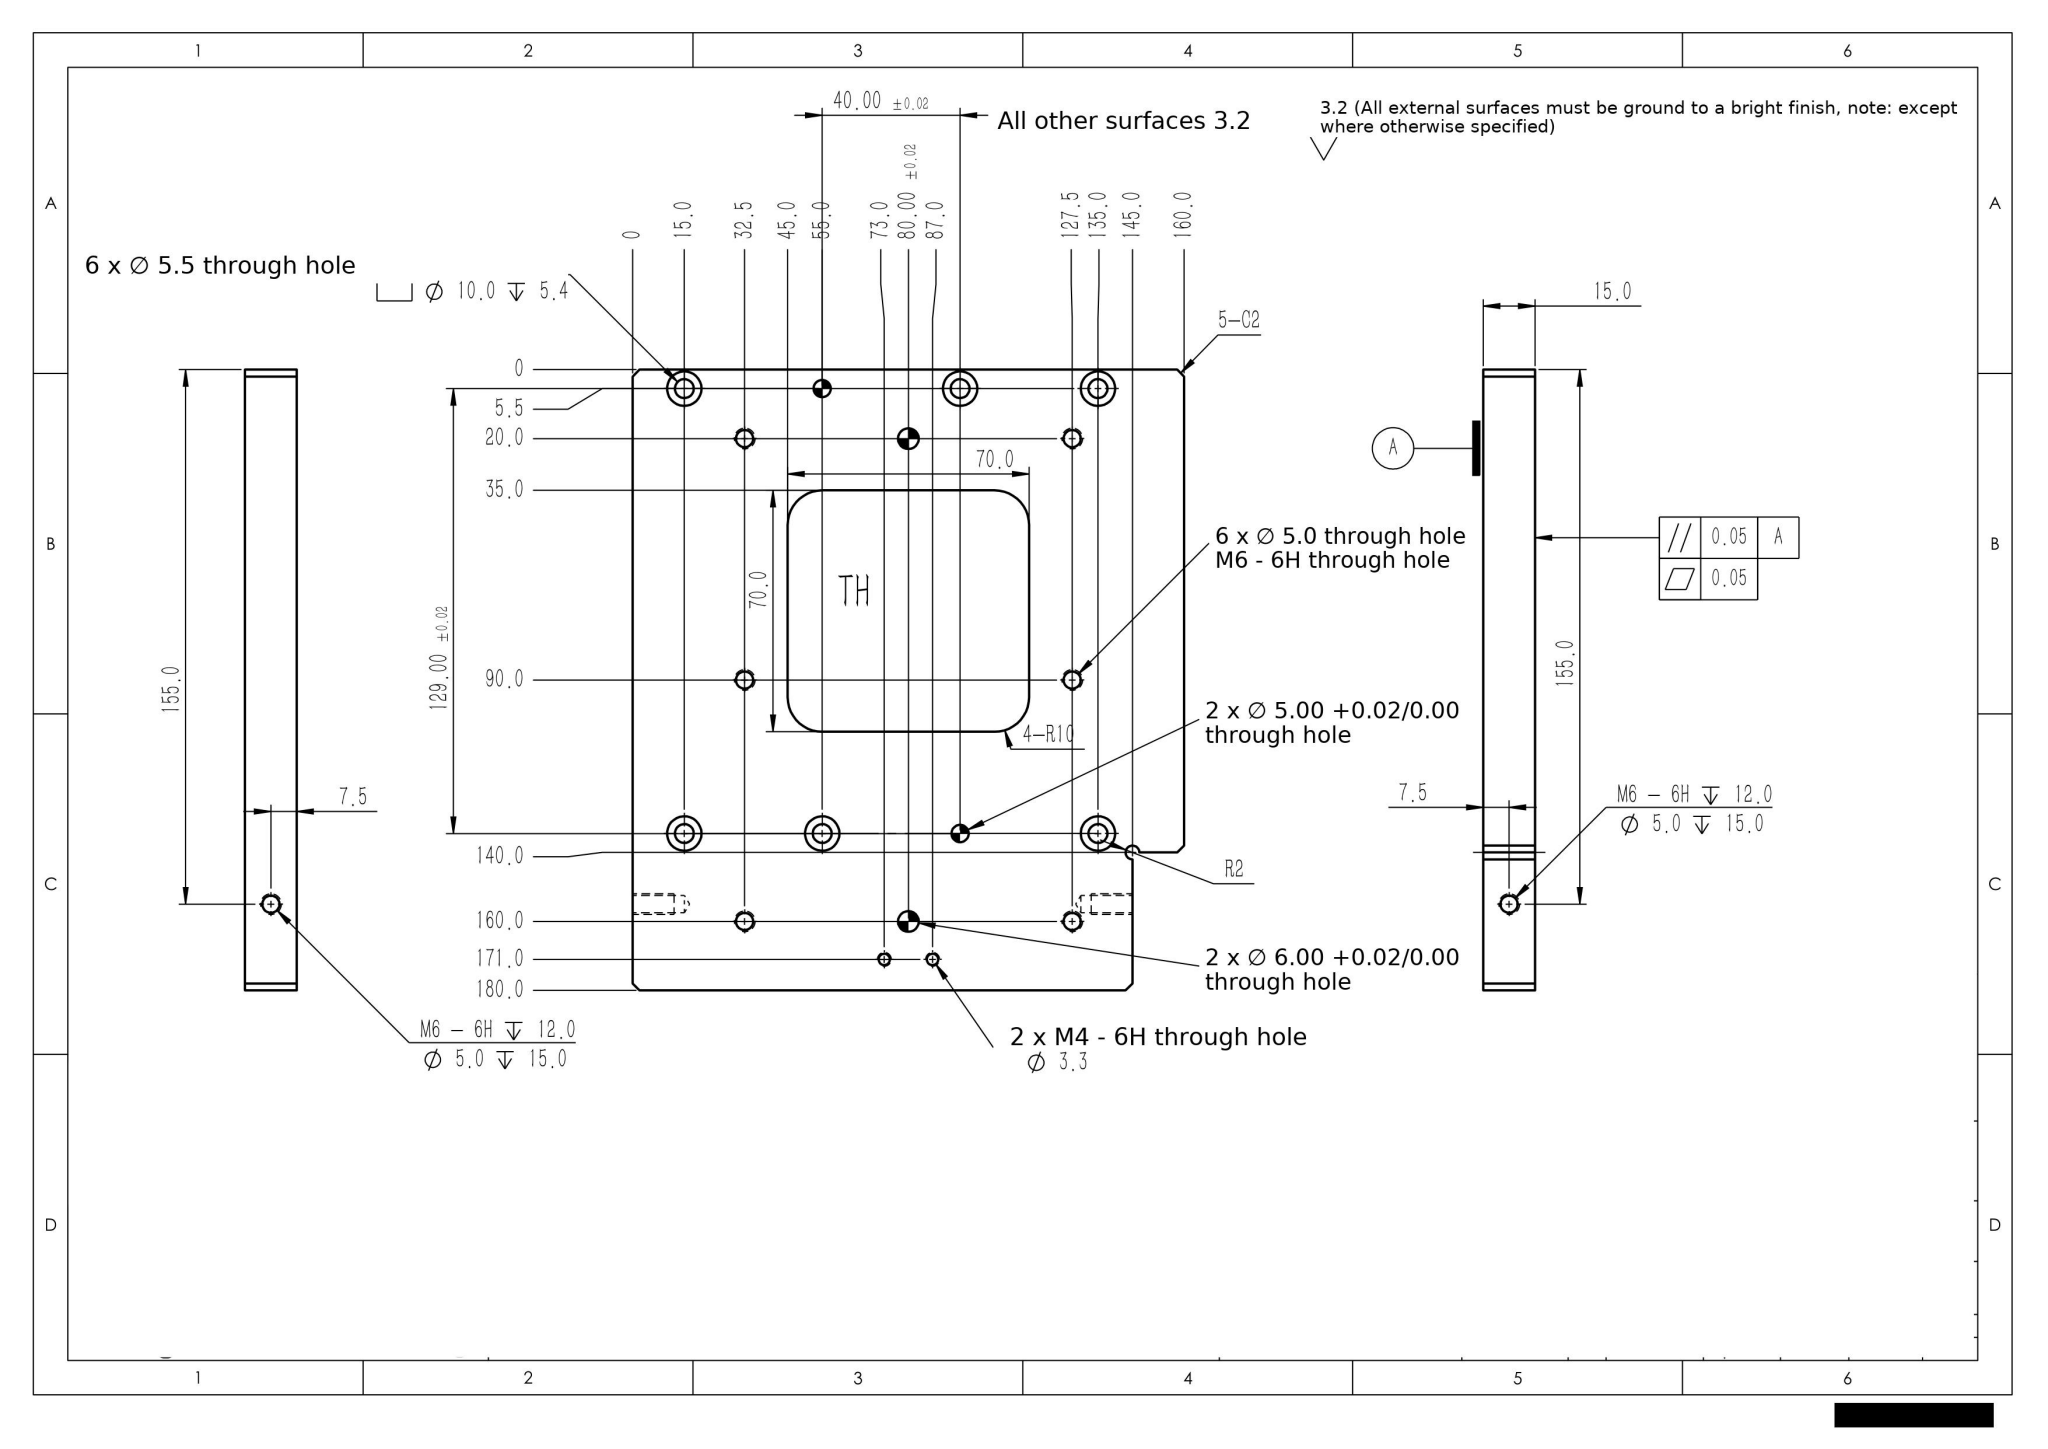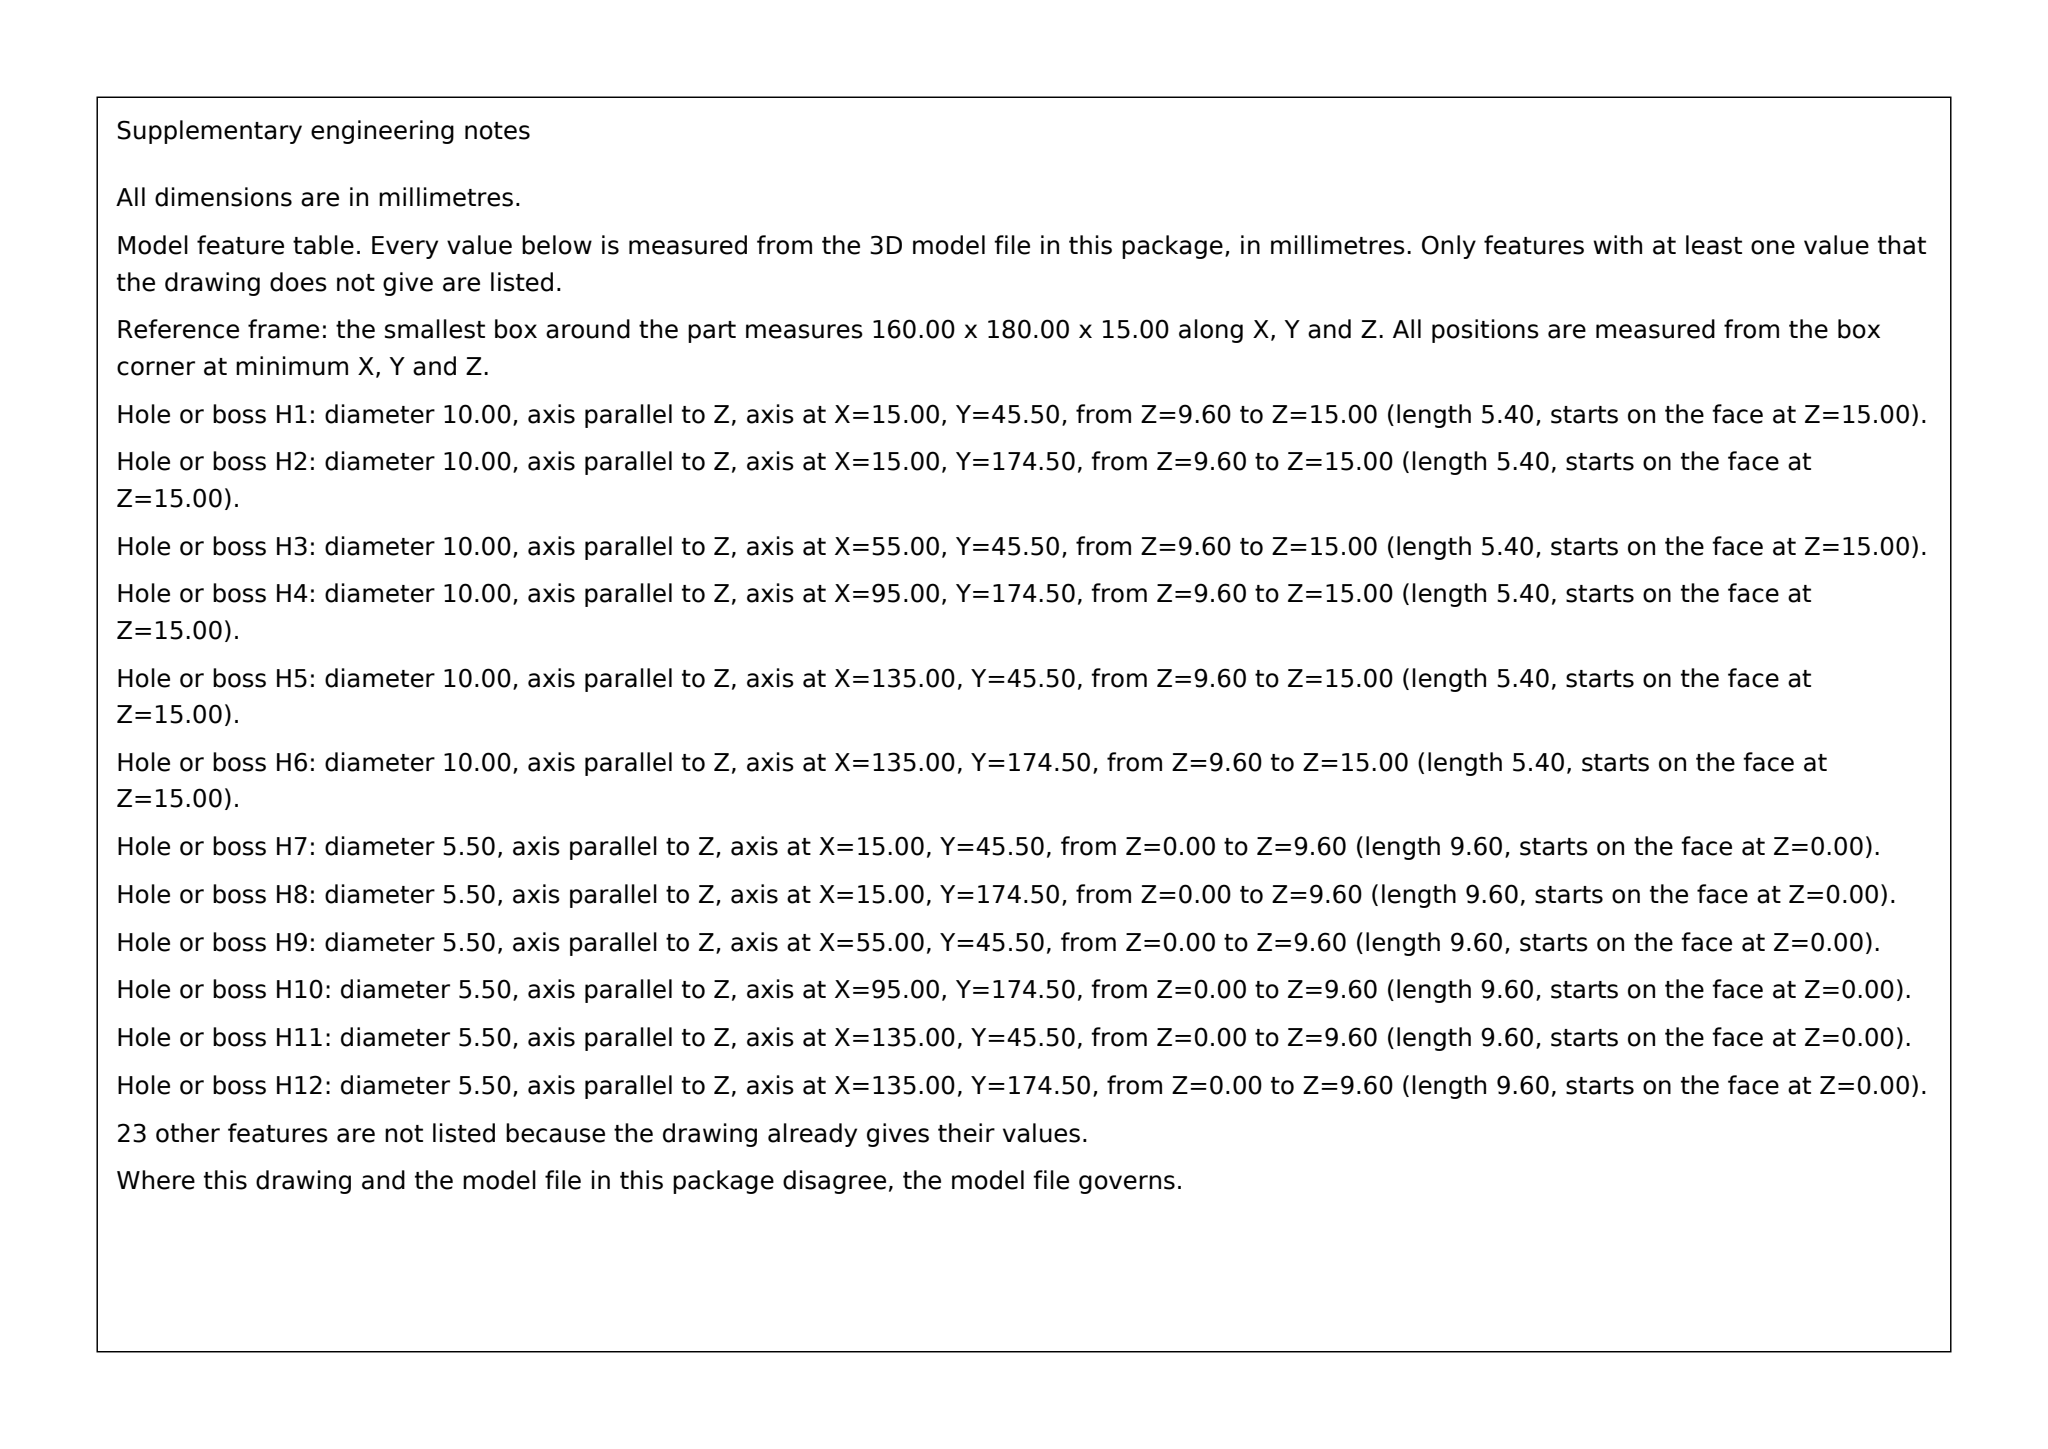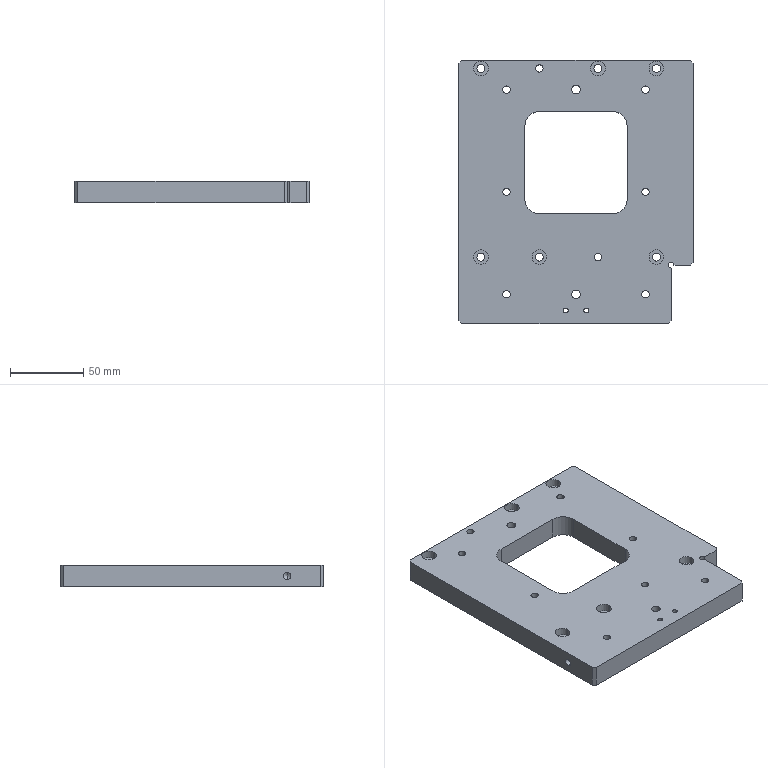Part | SolidWorks | mm | 1 solid | 84 faces | box 160 x 180 x 15 mm | volume 342513 mm3 | cylinder 57 | plane 23 | cone 4 | commonest cylinder face diameters 5 x20 10 x12 5.5 x12 3.3 x4 6 x4 20 x4 4 x1
build123d program:
from build123d import *

# Parameters (mm, degrees)
SKETCH1_W                                       = 160
SKETCH1_H                                       = 180
BOSS_EXTRUDE1_DEPTH                             = 15
M6_TAPPED_HOLE1_D                               = 5
SIZE_MM_DOWEL_PIN_HOLE_1_D                      = 6
M5_HEX_SOCKET_HEAD_CAP_SCREW_CBORE1_D           = 5.5
M5_HEX_SOCKET_HEAD_CAP_SCREW_CBORE1_CBORE_D     = 10
M5_HEX_SOCKET_HEAD_CAP_SCREW_CBORE1_CBORE_DEPTH = 5.4
SIZE_MM_DOWEL_PIN_HOLE_5_D                      = 5
SKETCH19_W                                      = 70
SKETCH19_H                                      = 70
CUT_EXTRUDE1_DEPTH                              = 122.347
FILLET1_R                                       = 10
SKETCH20_W                                      = 15
SKETCH20_H                                      = 40
CUT_EXTRUDE2_DEPTH                              = 122.347
M6_TAPPED_HOLE2_D                               = 5
M6_TAPPED_HOLE2_DEPTH                           = 15
M6_TAPPED_HOLE2_TIP                             = 1.502
CUT_EXTRUDE3_DEPTH                              = 122.347
CUT_EXTRUDE3_DEPTH_BACK                         = 122.347
SKETCH23_R                                      = 2
CHAMFER1_SIZE                                   = 2
M6_TAPPED_HOLE3_D                               = 5
M6_TAPPED_HOLE3_DEPTH                           = 15
M6_TAPPED_HOLE3_TIP                             = 1.502
M4_TAPPED_HOLE1_D                               = 3.3


with BuildPart() as part:
    # Sketch1 → Boss-Extrude1 (new body)
    with BuildSketch(Plane.XY):
        Rectangle(SKETCH1_W, SKETCH1_H)
    extrude(amount=BOSS_EXTRUDE1_DEPTH)

    # M6 Tapped Hole1 (through all)
    with Locations(Plane.XY.offset(15)):
        with Locations((-47.5, 70), (-47.5, -70), (47.5, 70), (47.5, -70), (-47.5, 0), (47.5, 0)):
            Hole(M6_TAPPED_HOLE1_D / 2)

    # Size mm Dowel Pin Hole 1 (through all)
    with Locations(Plane.XY.offset(15)):
        with Locations((0, 70), (0, -70)):
            Hole(SIZE_MM_DOWEL_PIN_HOLE_1_D / 2)

    # M5 Hex Socket Head Cap Screw CBORE1 (through all)
    with Locations(Plane.XY.offset(15)):
        with Locations((-65, 84.5), (15, 84.5), (55, 84.5), (-65, -44.5), (-25, -44.5), (55, -44.5)):
            CounterBoreHole(M5_HEX_SOCKET_HEAD_CAP_SCREW_CBORE1_D / 2, M5_HEX_SOCKET_HEAD_CAP_SCREW_CBORE1_CBORE_D / 2, M5_HEX_SOCKET_HEAD_CAP_SCREW_CBORE1_CBORE_DEPTH)

    # Size mm Dowel Pin Hole 5 (through all)
    with Locations(Plane.XY.offset(15)):
        with Locations((-25, 84.5), (15, -44.5)):
            Hole(SIZE_MM_DOWEL_PIN_HOLE_5_D / 2)

    # Sketch19 → Cut-Extrude1 (cut, through all)
    with BuildSketch(Plane.XY.offset(15)):
        with Locations((0, 20)):
            Rectangle(SKETCH19_W, SKETCH19_H)
    extrude(amount=-CUT_EXTRUDE1_DEPTH, mode=Mode.SUBTRACT)

    # Fillet1
    fillet1_edges = [part.edges().sort_by_distance(p)[0] for p in [
        (-35, -15, 7.5),
        (-35, 55, 7.5),
        (35, 55, 7.5),
        (35, -15, 7.5),
    ]]
    fillet(fillet1_edges, radius=FILLET1_R)

    # Sketch20 → Cut-Extrude2 (cut, through all)
    with BuildSketch(Plane.XY.offset(15)):
        with Locations((72.5, -70)):
            Rectangle(SKETCH20_W, SKETCH20_H)
    extrude(amount=-CUT_EXTRUDE2_DEPTH, mode=Mode.SUBTRACT)

    # M6 Tapped Hole2
    with Locations(Plane(origin=(65, 0, 0), x_dir=(0, 0, -1), z_dir=(1, 0, 0))):
        with Locations((-7.5, -65)):
            Hole(M6_TAPPED_HOLE2_D / 2, depth=M6_TAPPED_HOLE2_DEPTH)
            with Locations((0, 0, -(M6_TAPPED_HOLE2_DEPTH + M6_TAPPED_HOLE2_TIP / 2))):  # 118° drill point
                Cone(0, M6_TAPPED_HOLE2_D / 2, M6_TAPPED_HOLE2_TIP, mode=Mode.SUBTRACT)

    # Sketch23 → Cut-Extrude3 (cut, two sides: drawn at the far end of the back side and taken through both)
    with BuildSketch(Plane.XY.offset(15).offset(-CUT_EXTRUDE3_DEPTH_BACK)):
        with Locations((65, -50)):
            Circle(SKETCH23_R)
    extrude(amount=CUT_EXTRUDE3_DEPTH + CUT_EXTRUDE3_DEPTH_BACK, mode=Mode.SUBTRACT)

    # Chamfer1
    chamfer1_edges = [part.edges().sort_by_distance(p)[0] for p in [
        (80, -50, 7.5),
        (65, -90, 7.5),
        (-80, -90, 7.5),
        (-80, 90, 7.5),
        (80, 90, 7.5),
    ]]
    chamfer(chamfer1_edges, length=CHAMFER1_SIZE)

    # M6 Tapped Hole3
    with Locations(Plane.ZY.offset(80)):
        with Locations((7.5, -65)):
            Hole(M6_TAPPED_HOLE3_D / 2, depth=M6_TAPPED_HOLE3_DEPTH)
            with Locations((0, 0, -(M6_TAPPED_HOLE3_DEPTH + M6_TAPPED_HOLE3_TIP / 2))):  # 118° drill point
                Cone(0, M6_TAPPED_HOLE3_D / 2, M6_TAPPED_HOLE3_TIP, mode=Mode.SUBTRACT)

    # M4 Tapped Hole1 (through all)
    with Locations(Plane(origin=(0, 0, 0), x_dir=(-1, 0, 0), z_dir=(0, 0, -1))):
        with Locations((7, -81), (-7, -81)):
            Hole(M4_TAPPED_HOLE1_D / 2)


solid = part.part